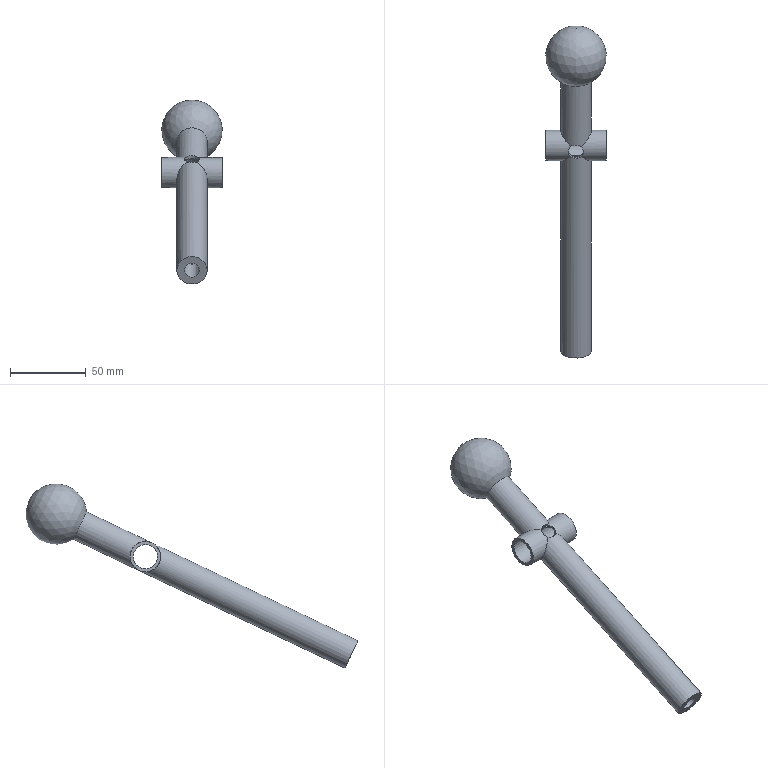Component | NX | HANDLE_ROD | 1 solid | 23 faces | volume 92585 mm3 | cylinder 9 | spline 6 | plane 6 | sphere 1 | cone 1 | commonest cylinder face diameters 20 x4 8.5 x2 10 x2 16 x1